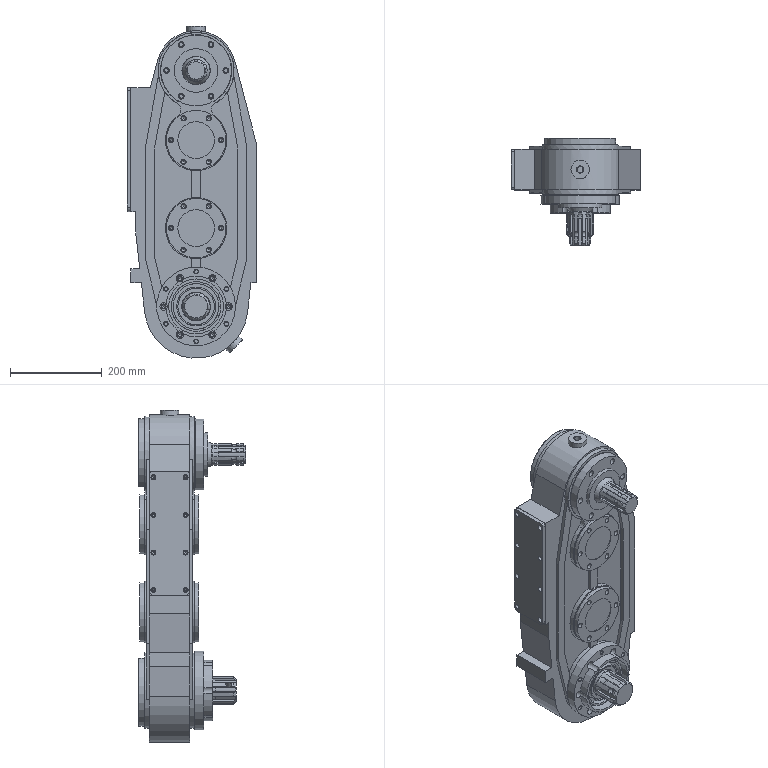Assembly | NX | mm | 26 component files | 26 solids | 1074 faces | box 283 x 234.25 x 725 mm | volume 8820590 mm3 | cylinder 410 | plane 353 | cone 267 | torus 42 | spline 2 | commonest cylinder face diameters 8.5 x54 12 x48 60 x38 11 x26 11.5 x24 51 x24 65 x16 50.5 x16
Bill of materials:
unnamed part 1 | 2 |  | Solid round flange plate with one straight flat cut along its edge, six through holes near the rim, and a raised circular boss on one face; no center bore is visible.
unnamed part 2 | 1 |  | Shaft with external straight splines along most of its length, a short collar or step partway along, a plain smaller-diameter round section at one end, and a small radial hole or notch near the other end.
unnamed part 3 | 1 |  | Ring-shaped flange with a large center bore, six through holes on a bolt circle, and a short hub on each face; the two hubs have different diameters.
unnamed part 4 | 1 |  | Thin flat gasket-like sheet with a roughly hexagonal outline, a rounded lobe at each of its six corners with a hole in each lobe, and a large circular center opening.
unnamed part 5 | 1 |  | Flange with a center bore, twelve through holes on a bolt circle, and a stepped hub on each face; one hub has internal stepped counterbores and scallop-shaped cutouts where it meets the bolt holes.
unnamed part 6 | 1 |  | Long housing or plate body with rounded ends, four large circular through bores in a row, a ring of small holes around each bore, small round bosses on the top and lower edges, and rectangular side extensions.
unnamed part 7 | 4 |  | Fully round solid flange plate with six through holes near the rim and a raised, chamfered circular boss on one face; no center bore is visible.
unnamed part 8 | 2 |  | Plain ring with a rectangular cross-section, flat faces, and plain inner and outer diameters.
unnamed part 9 | 4 |  | Thin flat annular sheet with a large center opening and six through holes evenly spaced around the band.
unnamed part 10 | 1 |  | Stepped shaft with two splined sections of different diameters joined by a tapered transition and a smooth middle section; it has a circumferential groove near the small end, a collar on the larger spline, and a plain round section at the far end.
unnamed part 11 | 2 |  | Solid cylindrical shaft with a central band of about eight raised external teeth or keys with chamfered ends; both shaft ends are chamfered.
unnamed part 12 | 2 |  | Plain flat ring with a rectangular cross-section; the radial band is wider than its thickness.
unnamed part 13 | 3 |  | Thin flat annular ring with a large central circular opening and six small circular through-holes evenly spaced around a bolt-circle; the outer circular edge has one straight chord-like flat cut across one side.
unnamed part 14 | 1 |  | Flat rectangular plate with slightly rounded corners and eight small circular through-holes arranged in two parallel rows of four along the long edges.
Mates:
1. touch align | oil_seal_85x60x8 1 face | oil_seal_85x60x8 2 face
2. touch align | oil_seal_85x60x8 1 face | oil_seal_85x60x8 2 face
3. touch align | oil_seal_85x60x8 1 face | end_cap2 1 face
4. touch align | oil_seal_85x60x8 1 face | end_cap2 1 face
5. touch align | T1_shim2 3 face | end_cap2 1 face
6. touch align | T1_shim2 3 face | end_cap2 1 face
7. touch align | T1_shim2 3 face | end_cap2 1 face
8. touch align | end_cap2 1 face | upper_shaft 1 face
9. touch align | upper_shaft 1 face | side_housing 1 face
10. touch align | end_cap2 1 face | side_housing 1 face
11. touch align | T1_shim2 2 face | end_cap3 2 face
12. touch align | T1_shim2 2 face | end_cap3 2 face
13. touch align | T1_shim2 2 face | end_cap3 2 face
14. touch align | end_cap3 2 face | side_housing 1 face
15. touch align | end_cap3 2 face | side_housing 1 face
16. touch align | T1_shim2 2 face | side_housing 1 face
17. fix | side_housing 1 component
18. touch align | T1_shim2 1 face | end_cap3 1 face
19. touch align | T1_shim2 1 face | end_cap3 1 face
20. touch align | T1_shim2 1 face | end_cap3 1 face
21. touch align | end_cap3 1 face | side_housing 1 face
22. touch align | end_cap3 1 face | side_housing 1 face
23. touch align | lower_end_cap 1 face | side_housing 1 face
24. touch align | lower_end_cap 1 face | side_housing 1 face
25. touch align | oil_seal_80x60x10 1 face | oil_seal_80x60x10 2 face
26. touch align | oil_seal_80x60x10 2 face | oil_seal_80x60x10 1 face
27. touch align | oil_seal_80x60x10 2 face | lower_end_cap 1 face
28. touch align | oil_seal_80x60x10 2 face | lower_end_cap 1 face
29. touch align | T1_shim3 1 face | lower_end_cap 1 face
30. touch align | T1_shim3 1 face | lower_end_cap 1 face
31. touch align | T1_shim3 1 face | lower_end_cap 1 face
32. touch align | lower_shaft 1 face | side_housing 1 face
33. touch align | T1_shim3 1 face | side_housing 1 face
34. touch align | T1_shim1 1 face | end_cap1 4 face
35. touch align | T1_shim1 4 face | end_cap1 3 face
36. touch align | T1_shim1 2 face | end_cap1 2 face
37. touch align | T1_shim1 3 face | end_cap1 1 face
38. touch align | T1_shim1 4 face | end_cap1 3 face
39. touch align | T1_shim1 4 face | end_cap1 3 face
40. touch align | T1_shim1 1 face | end_cap1 4 face
41. touch align | T1_shim1 1 face | end_cap1 4 face
42. touch align | T1_shim1 2 face | end_cap1 2 face
43. touch align | T1_shim1 2 face | end_cap1 2 face
44. touch align | T1_shim1 3 face | end_cap1 1 face
45. touch align | T1_shim1 3 face | end_cap1 1 face
46. touch align | end_cap1 2 face | side_housing 1 face
47. touch align | end_cap1 2 face | side_housing 1 face
48. touch align | end_cap1 1 face | side_housing 1 face
49. touch align | end_cap1 1 face | side_housing 1 face
50. touch align | end_cap1 4 face | side_housing 1 face
51. touch align | end_cap1 3 face | side_housing 1 face
52. touch align | end_cap1 3 face | side_housing 1 face
53. touch align | end_cap1 4 face | side_housing 1 face
54. touch align | T1_shim1 1 face | side_housing 1 face
55. touch align | T1_shim1 4 face | side_housing 1 face
56. touch align | housing_cover 1 face | side_housing 1 face
57. touch align | housing_cover 1 face | side_housing 1 face
58. touch align | housing_cover 1 face | side_housing 1 face